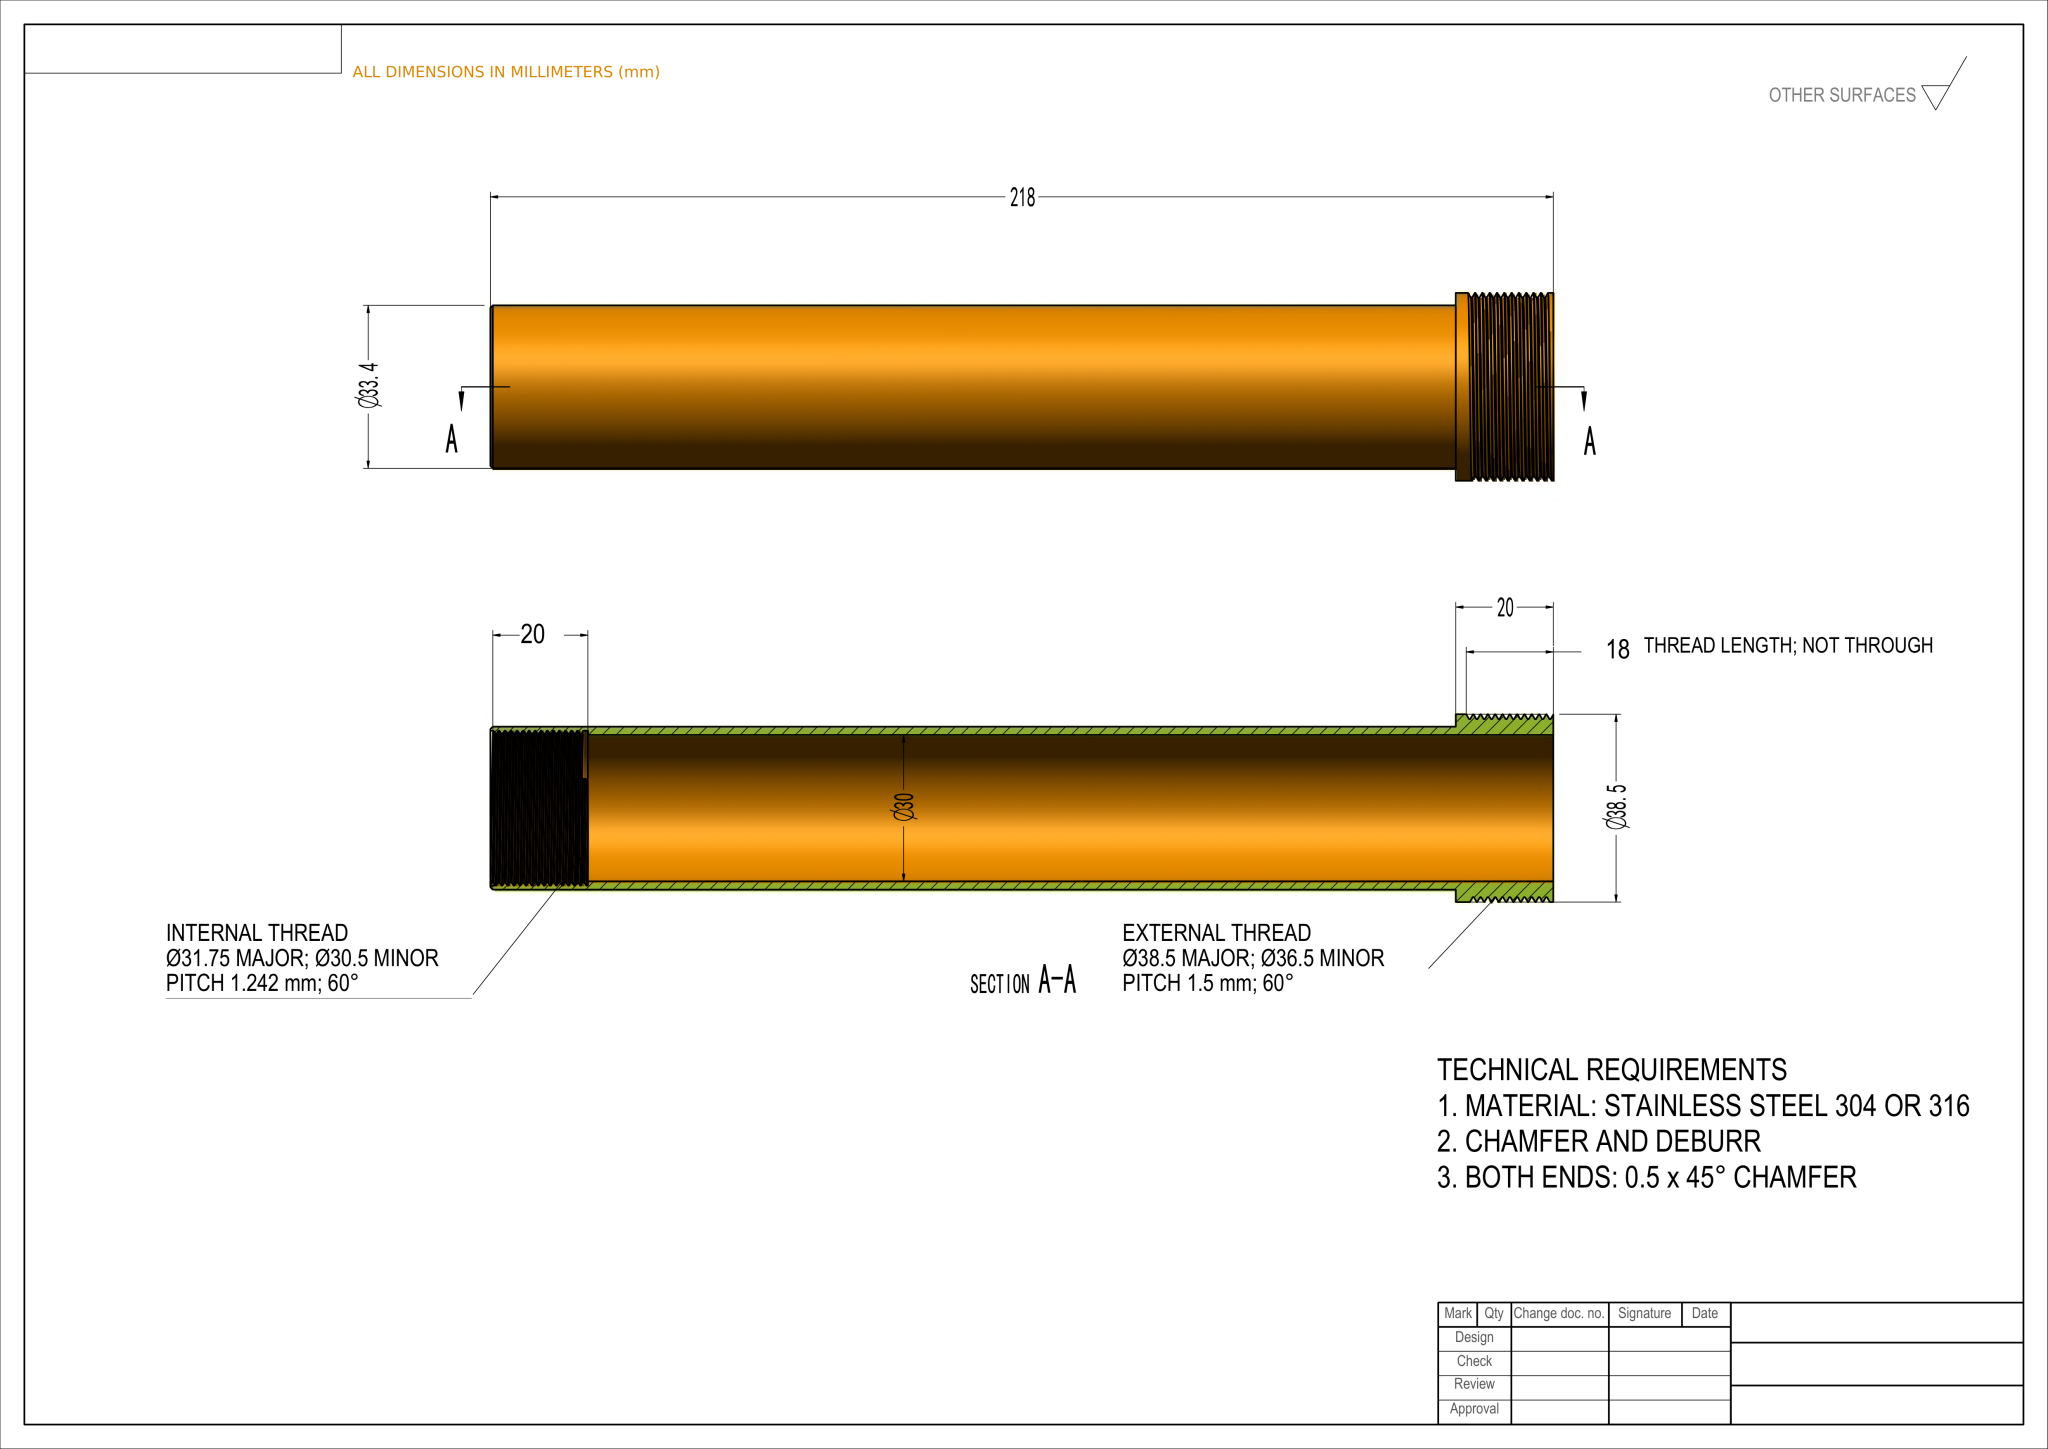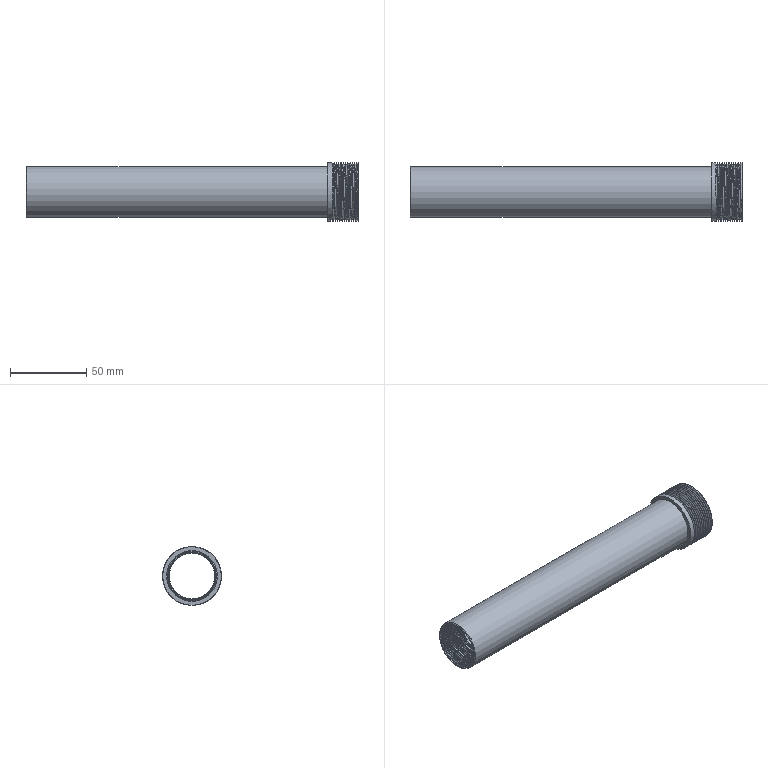Part | NX | mm | 1 solid | 30 faces | box 218 x 38.5 x 38.5 mm | volume 39915 mm3 | cylinder 17 | plane 8 | spline 4 | cone 1 | commonest cylinder face diameters 38.5 x12 33.4 x1 30.5 x1 31.75 x1 30 x1 36.5 x1